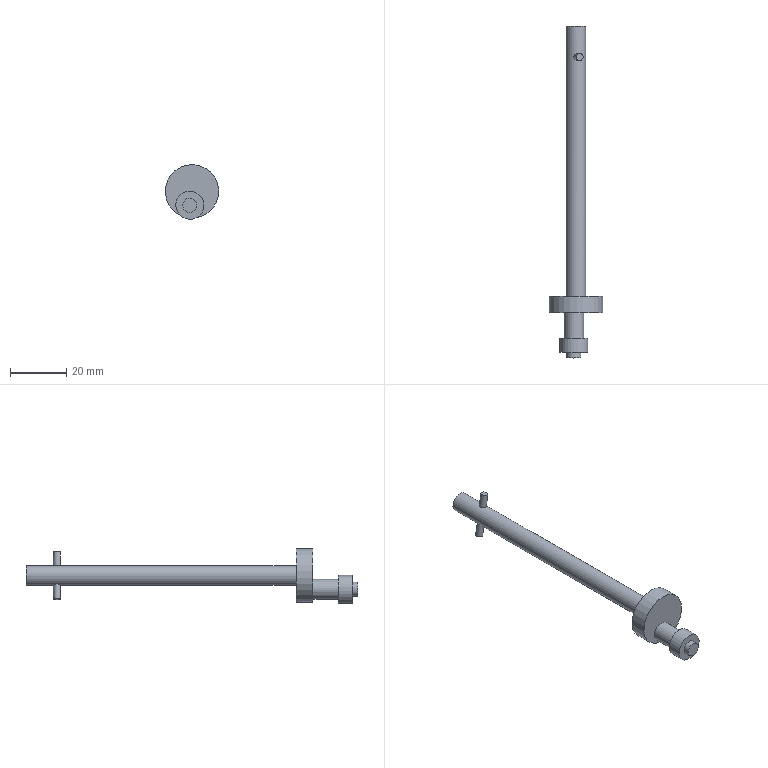Component | NX | LARGE_GEAR_SHAFT | 1 solid | 15 faces | volume 6224 mm3 | plane 8 | cylinder 7 | commonest cylinder face diameters 7 x2 2.5 x2 19 x1 10 x1 5 x1